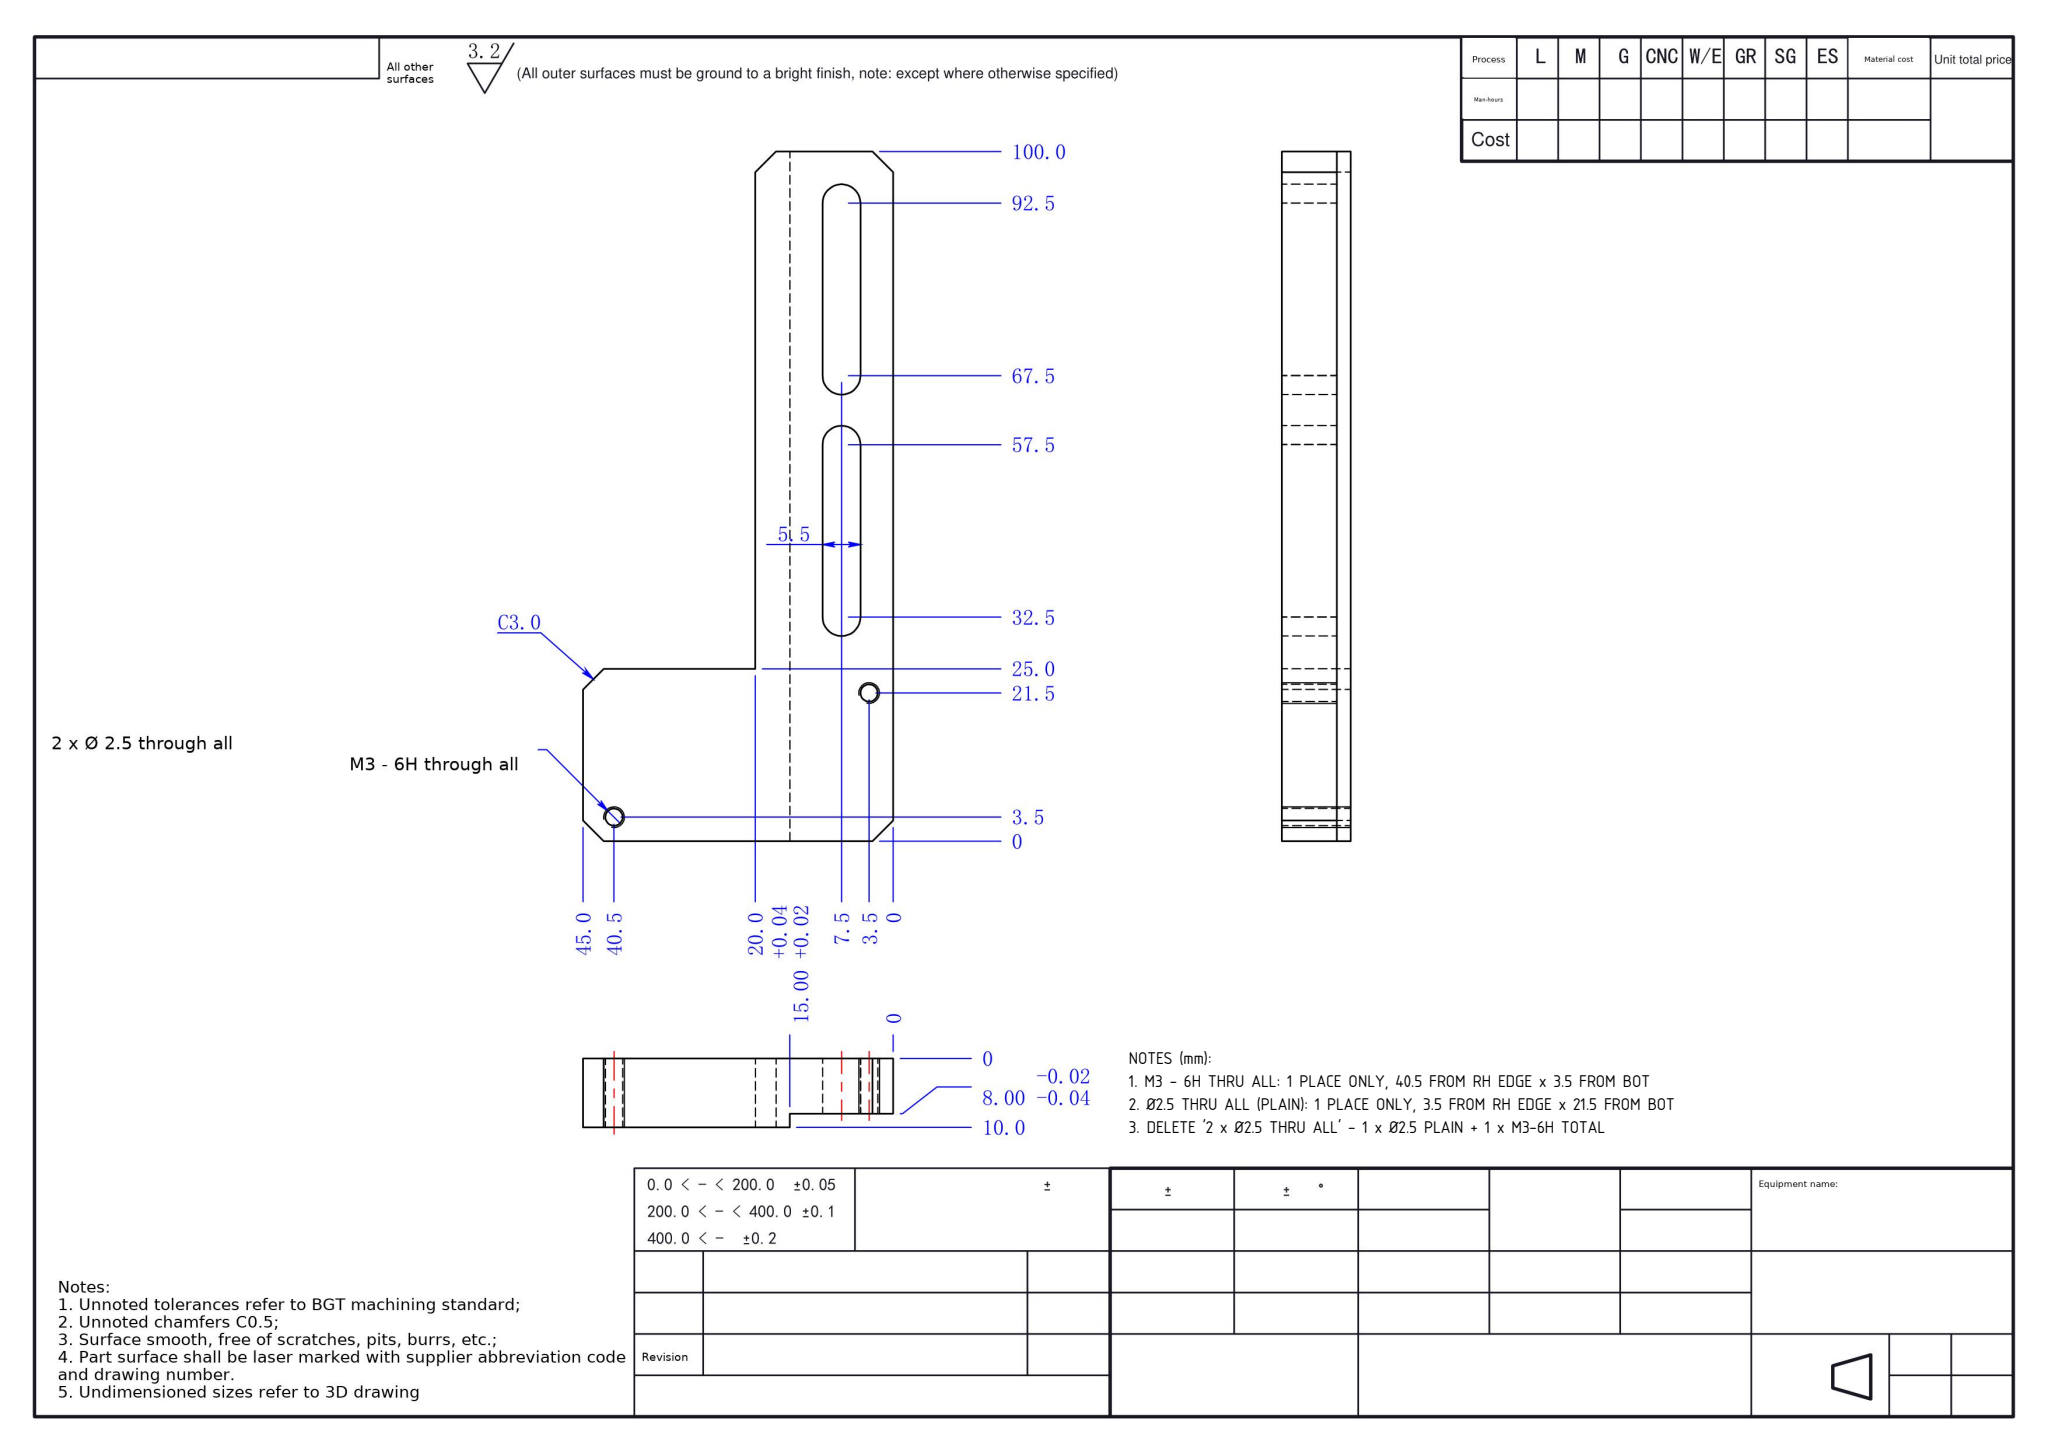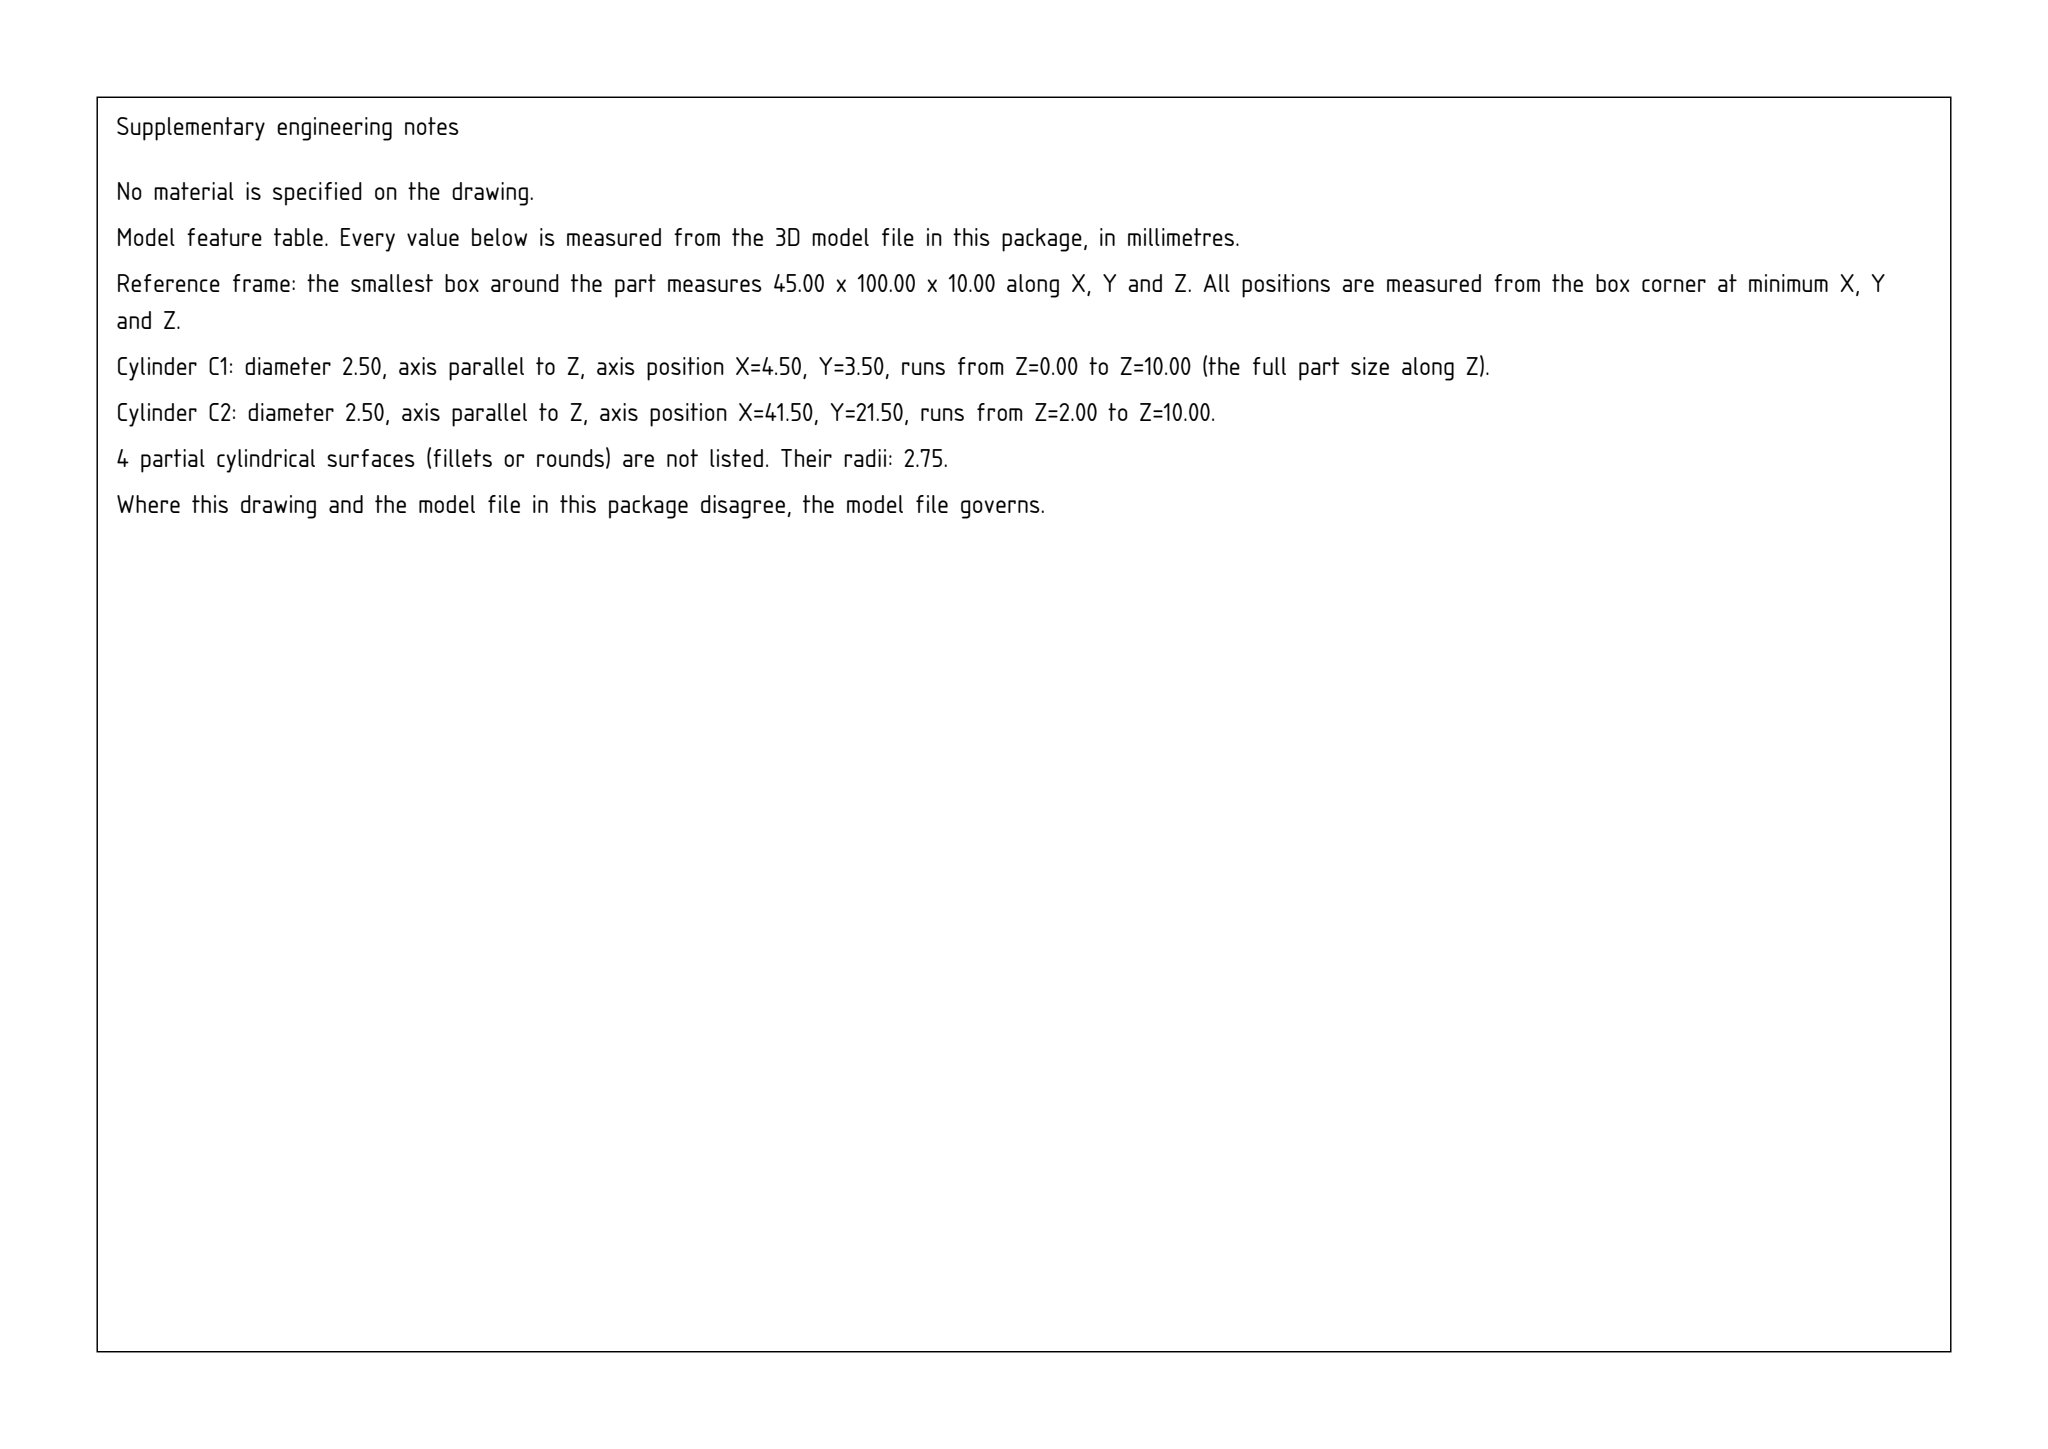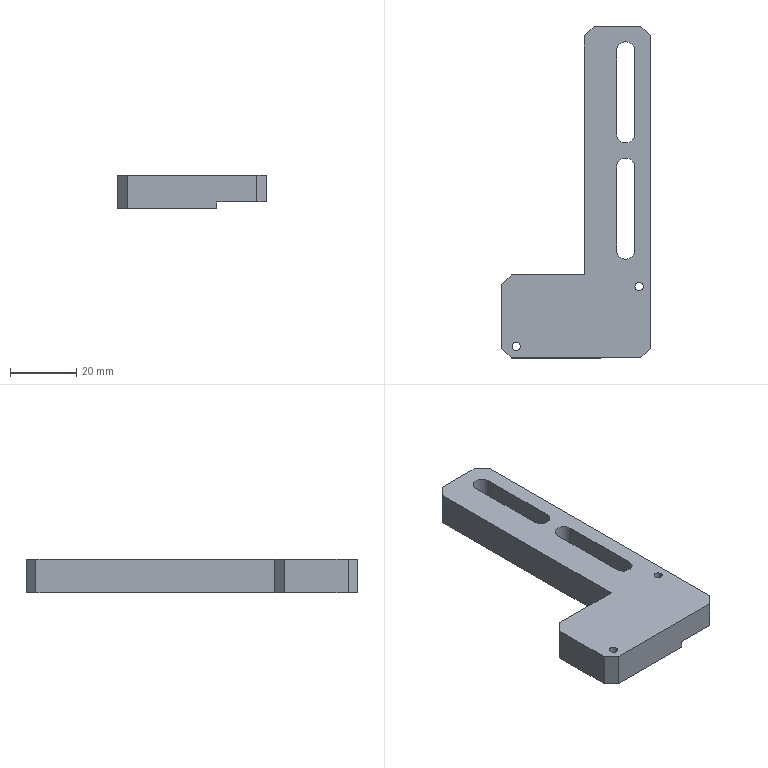Part | SolidWorks | mm | 1 solid | 27 faces | box 45 x 100 x 10 mm | volume 20375 mm3 | plane 19 | cylinder 8 | commonest cylinder face diameters 2.5 x4 5.5 x4
Drawing notes:
M3 - 6H THRU ALL: 1 PLACE ONLY, 40.5 FROM RH EDGE x 3.5 FROM BOT | from the solid: Ø2.5 z-axis cyl at (x=4.5, y=3.5), length 10 = full 10 thk; = 45.0-40.5 from RH edge datum (x=0 at right), 3.5 above y=0 bottom edge
Ø2.5 THRU ALL (PLAIN): 1 PLACE ONLY, 3.5 FROM RH EDGE x 21.5 FROM BOT | from the solid: Ø2.5 z-axis cyl at (x=41.5, y=21.5), length 8 = thk of 8.00 step region (z 2.0-10.0); = 45.0-41.5 from RH edge, 21.5 above bottom edge; only two Ø2.5 holes exist in model
DELETE '2 x Ø2.5 THRU ALL' - 1 x Ø2.5 PLAIN + 1 x M3-6H TOTAL | from the solid: Model contains exactly two Ø2.5 z-axis holes: (4.5,3.5) L10 and (41.5,21.5) L8
build123d program:
from build123d import *

# Parameters (mm, degrees)
SKETCH1_W           = 45
SKETCH1_H           = 100
BOSS_EXTRUDE1_DEPTH = 10
SKETCH2_W           = 25
SKETCH2_H           = 75
CUT_EXTRUDE1_DEPTH  = 111.114
SKETCH3_W           = 15
SKETCH3_H           = 100
CUT_EXTRUDE2_DEPTH  = 2
CHAMFER1_SIZE       = 3
CUT_EXTRUDE3_DEPTH  = 111.114
M3_TAPPED_HOLE1_D   = 2.5


with BuildPart() as part:
    # Sketch1 → Boss-Extrude1 (new body)
    with BuildSketch(Plane.XY):
        with Locations((22.5, 50)):
            Rectangle(SKETCH1_W, SKETCH1_H)
    extrude(amount=BOSS_EXTRUDE1_DEPTH)

    # Sketch2 → Cut-Extrude1 (cut, through all)
    with BuildSketch(Plane.XY.offset(10)):
        with Locations((12.5, 62.5)):
            Rectangle(SKETCH2_W, SKETCH2_H)
    extrude(amount=-CUT_EXTRUDE1_DEPTH, mode=Mode.SUBTRACT)

    # Sketch3 → Cut-Extrude2 (cut)
    with BuildSketch(Plane(origin=(0, 0, 0), x_dir=(-1, 0, 0), z_dir=(0, 0, -1))):
        with Locations((-37.5, 50)):
            Rectangle(SKETCH3_W, SKETCH3_H)
    extrude(amount=-CUT_EXTRUDE2_DEPTH, mode=Mode.SUBTRACT)

    # Chamfer1
    chamfer1_edges = [part.edges().sort_by_distance(p)[0] for p in [
        (0, 25, 5),
        (25, 100, 5),
        (45, 100, 6),
        (45, 0, 6),
        (0, 0, 5),
    ]]
    chamfer(chamfer1_edges, length=CHAMFER1_SIZE)

    # Sketch4 → Cut-Extrude3 (cut, through all)
    with BuildSketch(Plane.XY.offset(10)):
        with BuildLine():
            Line((40.25, 92.5), (40.25, 67.5))
            ThreePointArc((40.25, 67.5), (37.5, 64.75), (34.75, 67.5))
            Line((34.75, 67.5), (34.75, 92.5))
            ThreePointArc((34.75, 92.5), (37.5, 95.25), (40.25, 92.5))
        make_face()
        with BuildLine():
            Line((40.25, 57.5), (40.25, 32.5))
            ThreePointArc((40.25, 32.5), (37.5, 29.75), (34.75, 32.5))
            Line((34.75, 32.5), (34.75, 57.5))
            ThreePointArc((34.75, 57.5), (37.5, 60.25), (40.25, 57.5))
        make_face()
    extrude(amount=-CUT_EXTRUDE3_DEPTH, mode=Mode.SUBTRACT)

    # M3 Tapped Hole1 (through all)
    with Locations(Plane.XY.offset(10)):
        with Locations((4.5, 3.5), (41.5, 21.5)):
            Hole(M3_TAPPED_HOLE1_D / 2)


solid = part.part
STEP:
#1=CARTESIAN_POINT('',(3.25,3.5,0.));
#2=VERTEX_POINT('',#1);
#3=CARTESIAN_POINT('',(5.75,3.5,0.));
#4=VERTEX_POINT('',#3);
#5=CARTESIAN_POINT('',(4.5,3.5,0.));
#6=DIRECTION('',(0.,0.,1.));
#7=DIRECTION('',(1.,0.,0.));
#8=AXIS2_PLACEMENT_3D('',#5,#6,#7);
#9=CIRCLE('',#8,1.25);
#10=EDGE_CURVE('',#2,#4,#9,.T.);
#11=ORIENTED_EDGE('',*,*,#10,.F.);
#12=CARTESIAN_POINT('',(3.25,3.5,10.));
#13=VERTEX_POINT('',#12);
#14=CARTESIAN_POINT('',(3.25,3.5,10.));
#15=DIRECTION('',(0.,0.,1.));
#16=VECTOR('',#15,1000.);
#17=LINE('',#14,#16);
#18=EDGE_CURVE('',#2,#13,#17,.T.);
#19=ORIENTED_EDGE('',*,*,#18,.T.);
#20=CARTESIAN_POINT('',(5.75,3.5,10.));
#21=VERTEX_POINT('',#20);
#22=CARTESIAN_POINT('',(4.5,3.5,10.));
#23=DIRECTION('',(0.,0.,1.));
#24=DIRECTION('',(1.,0.,0.));
#25=AXIS2_PLACEMENT_3D('',#22,#23,#24);
#26=CIRCLE('',#25,1.25);
#27=EDGE_CURVE('',#13,#21,#26,.T.);
#28=ORIENTED_EDGE('',*,*,#27,.T.);
#29=CARTESIAN_POINT('',(5.75,3.5,10.));
#30=DIRECTION('',(0.,0.,1.));
#31=VECTOR('',#30,1000.);
#32=LINE('',#29,#31);
#33=EDGE_CURVE('',#4,#21,#32,.T.);
#34=ORIENTED_EDGE('',*,*,#33,.F.);
#35=EDGE_LOOP('',(#11,#19,#28,#34));
#36=FACE_OUTER_BOUND('',#35,.T.);
#37=CARTESIAN_POINT('',(4.5,3.5,10.));
#38=DIRECTION('',(0.,0.,1.));
#39=DIRECTION('',(1.,0.,0.));
#40=AXIS2_PLACEMENT_3D('',#37,#38,#39);
#41=CYLINDRICAL_SURFACE('',#40,1.25);
#42=ADVANCED_FACE('',(#36),#41,.F.);
#43=CARTESIAN_POINT('',(42.75,21.5,2.));
#44=VERTEX_POINT('',#43);
#45=CARTESIAN_POINT('',(40.25,21.5,2.));
#46=VERTEX_POINT('',#45);
#47=CARTESIAN_POINT('',(41.5,21.5,2.));
#48=DIRECTION('',(0.,0.,-1.));
#49=DIRECTION('',(-1.,0.,0.));
#50=AXIS2_PLACEMENT_3D('',#47,#48,#49);
#51=CIRCLE('',#50,1.25);
#52=EDGE_CURVE('',#44,#46,#51,.T.);
#53=ORIENTED_EDGE('',*,*,#52,.T.);
#54=CARTESIAN_POINT('',(40.25,21.5,10.));
#55=VERTEX_POINT('',#54);
#56=CARTESIAN_POINT('',(40.25,21.5,10.));
#57=DIRECTION('',(0.,0.,1.));
#58=VECTOR('',#57,1000.);
#59=LINE('',#56,#58);
#60=EDGE_CURVE('',#46,#55,#59,.T.);
#61=ORIENTED_EDGE('',*,*,#60,.T.);
#62=CARTESIAN_POINT('',(42.75,21.5,10.));
#63=VERTEX_POINT('',#62);
#64=CARTESIAN_POINT('',(41.5,21.5,10.));
#65=DIRECTION('',(0.,0.,1.));
#66=DIRECTION('',(1.,0.,0.));
#67=AXIS2_PLACEMENT_3D('',#64,#65,#66);
#68=CIRCLE('',#67,1.25);
#69=EDGE_CURVE('',#55,#63,#68,.T.);
#70=ORIENTED_EDGE('',*,*,#69,.T.);
#71=CARTESIAN_POINT('',(42.75,21.5,10.));
#72=DIRECTION('',(0.,0.,1.));
#73=VECTOR('',#72,1000.);
#74=LINE('',#71,#73);
#75=EDGE_CURVE('',#44,#63,#74,.T.);
#76=ORIENTED_EDGE('',*,*,#75,.F.);
#77=EDGE_LOOP('',(#53,#61,#70,#76));
#78=FACE_OUTER_BOUND('',#77,.T.);
#79=CARTESIAN_POINT('',(41.5,21.5,10.));
#80=DIRECTION('',(0.,0.,1.));
#81=DIRECTION('',(1.,0.,0.));
#82=AXIS2_PLACEMENT_3D('',#79,#80,#81);
#83=CYLINDRICAL_SURFACE('',#82,1.25);
#84=ADVANCED_FACE('',(#78),#83,.F.);
#85=CARTESIAN_POINT('',(41.5,21.5,10.));
#86=DIRECTION('',(0.,0.,1.));
#87=DIRECTION('',(1.,0.,0.));
#88=AXIS2_PLACEMENT_3D('',#85,#86,#87);
#89=CIRCLE('',#88,1.25);
#90=EDGE_CURVE('',#63,#55,#89,.T.);
#91=ORIENTED_EDGE('',*,*,#90,.F.);
#92=ORIENTED_EDGE('',*,*,#69,.F.);
#93=EDGE_LOOP('',(#91,#92));
#94=FACE_BOUND('',#93,.T.);
#95=CARTESIAN_POINT('',(34.75,57.5,10.));
#96=VERTEX_POINT('',#95);
#97=CARTESIAN_POINT('',(34.75,32.5,10.));
#98=VERTEX_POINT('',#97);
#99=CARTESIAN_POINT('',(34.75,57.5,10.));
#100=DIRECTION('',(0.,-1.,0.));
#101=VECTOR('',#100,1000.);
#102=LINE('',#99,#101);
#103=EDGE_CURVE('',#96,#98,#102,.T.);
#104=ORIENTED_EDGE('',*,*,#103,.F.);
#105=CARTESIAN_POINT('',(40.25,57.5,10.));
#106=VERTEX_POINT('',#105);
#107=CARTESIAN_POINT('',(37.5,57.5,10.));
#108=DIRECTION('',(0.,0.,1.));
#109=DIRECTION('',(1.,0.,0.));
#110=AXIS2_PLACEMENT_3D('',#107,#108,#109);
#111=CIRCLE('',#110,2.75);
#112=EDGE_CURVE('',#106,#96,#111,.T.);
#113=ORIENTED_EDGE('',*,*,#112,.F.);
#114=CARTESIAN_POINT('',(40.25,32.5,10.));
#115=VERTEX_POINT('',#114);
#116=CARTESIAN_POINT('',(40.25,57.5,10.));
#117=DIRECTION('',(-0.,1.,0.));
#118=VECTOR('',#117,1000.);
#119=LINE('',#116,#118);
#120=EDGE_CURVE('',#115,#106,#119,.T.);
#121=ORIENTED_EDGE('',*,*,#120,.F.);
#122=CARTESIAN_POINT('',(37.5,32.5,10.));
#123=DIRECTION('',(0.,0.,1.));
#124=DIRECTION('',(1.,0.,0.));
#125=AXIS2_PLACEMENT_3D('',#122,#123,#124);
#126=CIRCLE('',#125,2.75);
#127=EDGE_CURVE('',#98,#115,#126,.T.);
#128=ORIENTED_EDGE('',*,*,#127,.F.);
#129=EDGE_LOOP('',(#104,#113,#121,#128));
#130=FACE_BOUND('',#129,.T.);
#131=CARTESIAN_POINT('',(34.75,92.5,10.));
#132=VERTEX_POINT('',#131);
#133=CARTESIAN_POINT('',(34.75,67.5,10.));
#134=VERTEX_POINT('',#133);
#135=CARTESIAN_POINT('',(34.75,92.5,10.));
#136=DIRECTION('',(0.,-1.,0.));
#137=VECTOR('',#136,1000.);
#138=LINE('',#135,#137);
#139=EDGE_CURVE('',#132,#134,#138,.T.);
#140=ORIENTED_EDGE('',*,*,#139,.F.);
#141=CARTESIAN_POINT('',(40.25,92.5,10.));
#142=VERTEX_POINT('',#141);
#143=CARTESIAN_POINT('',(37.5,92.5,10.));
#144=DIRECTION('',(0.,0.,1.));
#145=DIRECTION('',(1.,0.,0.));
#146=AXIS2_PLACEMENT_3D('',#143,#144,#145);
#147=CIRCLE('',#146,2.75);
#148=EDGE_CURVE('',#142,#132,#147,.T.);
#149=ORIENTED_EDGE('',*,*,#148,.F.);
#150=CARTESIAN_POINT('',(40.25,67.5,10.));
#151=VERTEX_POINT('',#150);
#152=CARTESIAN_POINT('',(40.25,92.5,10.));
#153=DIRECTION('',(0.,1.,0.));
#154=VECTOR('',#153,1000.);
#155=LINE('',#152,#154);
#156=EDGE_CURVE('',#151,#142,#155,.T.);
#157=ORIENTED_EDGE('',*,*,#156,.F.);
#158=CARTESIAN_POINT('',(37.5,67.5,10.));
#159=DIRECTION('',(0.,0.,1.));
#160=DIRECTION('',(1.,0.,0.));
#161=AXIS2_PLACEMENT_3D('',#158,#159,#160);
#162=CIRCLE('',#161,2.75);
#163=EDGE_CURVE('',#134,#151,#162,.T.);
#164=ORIENTED_EDGE('',*,*,#163,.F.);
#165=EDGE_LOOP('',(#140,#149,#157,#164));
#166=FACE_BOUND('',#165,.T.);
#167=CARTESIAN_POINT('',(3.,0.,10.));
#168=VERTEX_POINT('',#167);
#169=CARTESIAN_POINT('',(42.,0.,10.));
#170=VERTEX_POINT('',#169);
#171=CARTESIAN_POINT('',(0.,0.,10.));
#172=DIRECTION('',(1.,0.,0.));
#173=VECTOR('',#172,1000.);
#174=LINE('',#171,#173);
#175=EDGE_CURVE('',#168,#170,#174,.T.);
#176=ORIENTED_EDGE('',*,*,#175,.T.);
#177=CARTESIAN_POINT('',(45.,3.,10.));
#178=VERTEX_POINT('',#177);
#179=CARTESIAN_POINT('',(45.,3.,10.));
#180=DIRECTION('',(0.7071,0.7071,0.));
#181=VECTOR('',#180,1000.);
#182=LINE('',#179,#181);
#183=EDGE_CURVE('',#170,#178,#182,.T.);
#184=ORIENTED_EDGE('',*,*,#183,.T.);
#185=CARTESIAN_POINT('',(45.,97.,10.));
#186=VERTEX_POINT('',#185);
#187=CARTESIAN_POINT('',(45.,0.,10.));
#188=DIRECTION('',(0.,1.,0.));
#189=VECTOR('',#188,1000.);
#190=LINE('',#187,#189);
#191=EDGE_CURVE('',#178,#186,#190,.T.);
#192=ORIENTED_EDGE('',*,*,#191,.T.);
#193=CARTESIAN_POINT('',(42.,100.,10.));
#194=VERTEX_POINT('',#193);
#195=CARTESIAN_POINT('',(42.,100.,10.));
#196=DIRECTION('',(-0.7071,0.7071,0.));
#197=VECTOR('',#196,1000.);
#198=LINE('',#195,#197);
#199=EDGE_CURVE('',#186,#194,#198,.T.);
#200=ORIENTED_EDGE('',*,*,#199,.T.);
#201=CARTESIAN_POINT('',(28.,100.,10.));
#202=VERTEX_POINT('',#201);
#203=CARTESIAN_POINT('',(0.,100.,10.));
#204=DIRECTION('',(-1.,0.,0.));
#205=VECTOR('',#204,1000.);
#206=LINE('',#203,#205);
#207=EDGE_CURVE('',#194,#202,#206,.T.);
#208=ORIENTED_EDGE('',*,*,#207,.T.);
#209=CARTESIAN_POINT('',(25.,97.,10.));
#210=VERTEX_POINT('',#209);
#211=CARTESIAN_POINT('',(28.,100.,10.));
#212=DIRECTION('',(-0.7071,-0.7071,0.));
#213=VECTOR('',#212,1000.);
#214=LINE('',#211,#213);
#215=EDGE_CURVE('',#202,#210,#214,.T.);
#216=ORIENTED_EDGE('',*,*,#215,.T.);
#217=CARTESIAN_POINT('',(25.,25.,10.));
#218=VERTEX_POINT('',#217);
#219=CARTESIAN_POINT('',(25.,100.,10.));
#220=DIRECTION('',(-0.,1.,0.));
#221=VECTOR('',#220,1000.);
#222=LINE('',#219,#221);
#223=EDGE_CURVE('',#218,#210,#222,.T.);
#224=ORIENTED_EDGE('',*,*,#223,.F.);
#225=CARTESIAN_POINT('',(3.,25.,10.));
#226=VERTEX_POINT('',#225);
#227=CARTESIAN_POINT('',(0.,25.,10.));
#228=DIRECTION('',(1.,0.,0.));
#229=VECTOR('',#228,1000.);
#230=LINE('',#227,#229);
#231=EDGE_CURVE('',#226,#218,#230,.T.);
#232=ORIENTED_EDGE('',*,*,#231,.F.);
#233=CARTESIAN_POINT('',(0.,22.,10.));
#234=VERTEX_POINT('',#233);
#235=CARTESIAN_POINT('',(3.,25.,10.));
#236=DIRECTION('',(-0.7071,-0.7071,0.));
#237=VECTOR('',#236,1000.);
#238=LINE('',#235,#237);
#239=EDGE_CURVE('',#226,#234,#238,.T.);
#240=ORIENTED_EDGE('',*,*,#239,.T.);
#241=CARTESIAN_POINT('',(0.,3.,10.));
#242=VERTEX_POINT('',#241);
#243=CARTESIAN_POINT('',(0.,0.,10.));
#244=DIRECTION('',(0.,-1.,0.));
#245=VECTOR('',#244,1000.);
#246=LINE('',#243,#245);
#247=EDGE_CURVE('',#234,#242,#246,.T.);
#248=ORIENTED_EDGE('',*,*,#247,.T.);
#249=CARTESIAN_POINT('',(3.,0.,10.));
#250=DIRECTION('',(0.7071,-0.7071,0.));
#251=VECTOR('',#250,1000.);
#252=LINE('',#249,#251);
#253=EDGE_CURVE('',#242,#168,#252,.T.);
#254=ORIENTED_EDGE('',*,*,#253,.T.);
#255=EDGE_LOOP('',(#176,#184,#192,#200,#208,#216,#224,#232,#240,#248,#254));
#256=FACE_OUTER_BOUND('',#255,.T.);
#257=CARTESIAN_POINT('',(4.5,3.5,10.));
#258=DIRECTION('',(0.,0.,1.));
#259=DIRECTION('',(1.,0.,0.));
#260=AXIS2_PLACEMENT_3D('',#257,#258,#259);
#261=CIRCLE('',#260,1.25);
#262=EDGE_CURVE('',#21,#13,#261,.T.);
#263=ORIENTED_EDGE('',*,*,#262,.F.);
#264=ORIENTED_EDGE('',*,*,#27,.F.);
#265=EDGE_LOOP('',(#263,#264));
#266=FACE_BOUND('',#265,.T.);
#267=CARTESIAN_POINT('',(0.,0.,10.));
#268=DIRECTION('',(0.,0.,-1.));
#269=DIRECTION('',(-1.,0.,0.));
#270=AXIS2_PLACEMENT_3D('',#267,#268,#269);
#271=PLANE('',#270);
#272=ADVANCED_FACE('',(#94,#130,#166,#256,#266),#271,.F.);
#273=ORIENTED_EDGE('',*,*,#191,.F.);
#274=CARTESIAN_POINT('',(45.,3.,2.));
#275=VERTEX_POINT('',#274);
#276=CARTESIAN_POINT('',(45.,3.,10.));
#277=DIRECTION('',(0.,0.,-1.));
#278=VECTOR('',#277,1000.);
#279=LINE('',#276,#278);
#280=EDGE_CURVE('',#178,#275,#279,.T.);
#281=ORIENTED_EDGE('',*,*,#280,.T.);
#282=CARTESIAN_POINT('',(45.,97.,2.));
#283=VERTEX_POINT('',#282);
#284=CARTESIAN_POINT('',(45.,100.,2.));
#285=DIRECTION('',(0.,-1.,0.));
#286=VECTOR('',#285,1000.);
#287=LINE('',#284,#286);
#288=EDGE_CURVE('',#283,#275,#287,.T.);
#289=ORIENTED_EDGE('',*,*,#288,.F.);
#290=CARTESIAN_POINT('',(45.,97.,10.));
#291=DIRECTION('',(0.,0.,1.));
#292=VECTOR('',#291,1000.);
#293=LINE('',#290,#292);
#294=EDGE_CURVE('',#283,#186,#293,.T.);
#295=ORIENTED_EDGE('',*,*,#294,.T.);
#296=EDGE_LOOP('',(#273,#281,#289,#295));
#297=FACE_OUTER_BOUND('',#296,.T.);
#298=CARTESIAN_POINT('',(45.,0.,10.));
#299=DIRECTION('',(-1.,0.,0.));
#300=DIRECTION('',(0.,0.,1.));
#301=AXIS2_PLACEMENT_3D('',#298,#299,#300);
#302=PLANE('',#301);
#303=ADVANCED_FACE('',(#297),#302,.F.);
#304=CARTESIAN_POINT('',(0.,22.,0.));
#305=VERTEX_POINT('',#304);
#306=CARTESIAN_POINT('',(0.,3.,0.));
#307=VERTEX_POINT('',#306);
#308=CARTESIAN_POINT('',(0.,0.,0.));
#309=DIRECTION('',(0.,-1.,0.));
#310=VECTOR('',#309,1000.);
#311=LINE('',#308,#310);
#312=EDGE_CURVE('',#305,#307,#311,.T.);
#313=ORIENTED_EDGE('',*,*,#312,.T.);
#314=CARTESIAN_POINT('',(0.,3.,10.));
#315=DIRECTION('',(0.,0.,1.));
#316=VECTOR('',#315,1000.);
#317=LINE('',#314,#316);
#318=EDGE_CURVE('',#307,#242,#317,.T.);
#319=ORIENTED_EDGE('',*,*,#318,.T.);
#320=ORIENTED_EDGE('',*,*,#247,.F.);
#321=CARTESIAN_POINT('',(0.,22.,10.));
#322=DIRECTION('',(0.,0.,-1.));
#323=VECTOR('',#322,1000.);
#324=LINE('',#321,#323);
#325=EDGE_CURVE('',#234,#305,#324,.T.);
#326=ORIENTED_EDGE('',*,*,#325,.T.);
#327=EDGE_LOOP('',(#313,#319,#320,#326));
#328=FACE_OUTER_BOUND('',#327,.T.);
#329=CARTESIAN_POINT('',(0.,0.,10.));
#330=DIRECTION('',(1.,0.,0.));
#331=DIRECTION('',(0.,0.,-1.));
#332=AXIS2_PLACEMENT_3D('',#329,#330,#331);
#333=PLANE('',#332);
#334=ADVANCED_FACE('',(#328),#333,.F.);
#335=CARTESIAN_POINT('',(42.,0.,2.));
#336=VERTEX_POINT('',#335);
#337=CARTESIAN_POINT('',(30.,0.,2.));
#338=VERTEX_POINT('',#337);
#339=CARTESIAN_POINT('',(45.,0.,2.));
#340=DIRECTION('',(-1.,0.,0.));
#341=VECTOR('',#340,1000.);
#342=LINE('',#339,#341);
#343=EDGE_CURVE('',#336,#338,#342,.T.);
#344=ORIENTED_EDGE('',*,*,#343,.F.);
#345=CARTESIAN_POINT('',(42.,0.,10.));
#346=DIRECTION('',(0.,0.,1.));
#347=VECTOR('',#346,1000.);
#348=LINE('',#345,#347);
#349=EDGE_CURVE('',#336,#170,#348,.T.);
#350=ORIENTED_EDGE('',*,*,#349,.T.);
#351=ORIENTED_EDGE('',*,*,#175,.F.);
#352=CARTESIAN_POINT('',(3.,0.,0.));
#353=VERTEX_POINT('',#352);
#354=CARTESIAN_POINT('',(3.,0.,10.));
#355=DIRECTION('',(0.,0.,-1.));
#356=VECTOR('',#355,1000.);
#357=LINE('',#354,#356);
#358=EDGE_CURVE('',#168,#353,#357,.T.);
#359=ORIENTED_EDGE('',*,*,#358,.T.);
#360=CARTESIAN_POINT('',(30.,0.,0.));
#361=VERTEX_POINT('',#360);
#362=CARTESIAN_POINT('',(0.,0.,0.));
#363=DIRECTION('',(1.,0.,0.));
#364=VECTOR('',#363,1000.);
#365=LINE('',#362,#364);
#366=EDGE_CURVE('',#353,#361,#365,.T.);
#367=ORIENTED_EDGE('',*,*,#366,.T.);
#368=CARTESIAN_POINT('',(30.,0.,2.));
#369=DIRECTION('',(0.,0.,-1.));
#370=VECTOR('',#369,1000.);
#371=LINE('',#368,#370);
#372=EDGE_CURVE('',#338,#361,#371,.T.);
#373=ORIENTED_EDGE('',*,*,#372,.F.);
#374=EDGE_LOOP('',(#344,#350,#351,#359,#367,#373));
#375=FACE_OUTER_BOUND('',#374,.T.);
#376=CARTESIAN_POINT('',(0.,0.,10.));
#377=DIRECTION('',(0.,1.,0.));
#378=DIRECTION('',(0.,0.,1.));
#379=AXIS2_PLACEMENT_3D('',#376,#377,#378);
#380=PLANE('',#379);
#381=ADVANCED_FACE('',(#375),#380,.F.);
#382=CARTESIAN_POINT('',(30.,100.,0.));
#383=VERTEX_POINT('',#382);
#384=CARTESIAN_POINT('',(28.,100.,0.));
#385=VERTEX_POINT('',#384);
#386=CARTESIAN_POINT('',(0.,100.,0.));
#387=DIRECTION('',(-1.,0.,0.));
#388=VECTOR('',#387,1000.);
#389=LINE('',#386,#388);
#390=EDGE_CURVE('',#383,#385,#389,.T.);
#391=ORIENTED_EDGE('',*,*,#390,.T.);
#392=CARTESIAN_POINT('',(28.,100.,10.));
#393=DIRECTION('',(0.,0.,1.));
#394=VECTOR('',#393,1000.);
#395=LINE('',#392,#394);
#396=EDGE_CURVE('',#385,#202,#395,.T.);
#397=ORIENTED_EDGE('',*,*,#396,.T.);
#398=ORIENTED_EDGE('',*,*,#207,.F.);
#399=CARTESIAN_POINT('',(42.,100.,2.));
#400=VERTEX_POINT('',#399);
#401=CARTESIAN_POINT('',(42.,100.,10.));
#402=DIRECTION('',(0.,0.,-1.));
#403=VECTOR('',#402,1000.);
#404=LINE('',#401,#403);
#405=EDGE_CURVE('',#194,#400,#404,.T.);
#406=ORIENTED_EDGE('',*,*,#405,.T.);
#407=CARTESIAN_POINT('',(30.,100.,2.));
#408=VERTEX_POINT('',#407);
#409=CARTESIAN_POINT('',(45.,100.,2.));
#410=DIRECTION('',(1.,0.,0.));
#411=VECTOR('',#410,1000.);
#412=LINE('',#409,#411);
#413=EDGE_CURVE('',#408,#400,#412,.T.);
#414=ORIENTED_EDGE('',*,*,#413,.F.);
#415=CARTESIAN_POINT('',(30.,100.,2.));
#416=DIRECTION('',(0.,0.,-1.));
#417=VECTOR('',#416,1000.);
#418=LINE('',#415,#417);
#419=EDGE_CURVE('',#408,#383,#418,.T.);
#420=ORIENTED_EDGE('',*,*,#419,.T.);
#421=EDGE_LOOP('',(#391,#397,#398,#406,#414,#420));
#422=FACE_OUTER_BOUND('',#421,.T.);
#423=CARTESIAN_POINT('',(0.,100.,10.));
#424=DIRECTION('',(0.,-1.,0.));
#425=DIRECTION('',(0.,0.,-1.));
#426=AXIS2_PLACEMENT_3D('',#423,#424,#425);
#427=PLANE('',#426);
#428=ADVANCED_FACE('',(#422),#427,.F.);
#429=CARTESIAN_POINT('',(4.5,3.5,0.));
#430=DIRECTION('',(0.,0.,1.));
#431=DIRECTION('',(1.,0.,0.));
#432=AXIS2_PLACEMENT_3D('',#429,#430,#431);
#433=CIRCLE('',#432,1.25);
#434=EDGE_CURVE('',#4,#2,#433,.T.);
#435=ORIENTED_EDGE('',*,*,#434,.T.);
#436=ORIENTED_EDGE('',*,*,#10,.T.);
#437=EDGE_LOOP('',(#435,#436));
#438=FACE_BOUND('',#437,.T.);
#439=ORIENTED_EDGE('',*,*,#366,.F.);
#440=CARTESIAN_POINT('',(1.5,1.5,0.));
#441=DIRECTION('',(-0.7071,0.7071,0.));
#442=VECTOR('',#441,1000.);
#443=LINE('',#440,#442);
#444=EDGE_CURVE('',#353,#307,#443,.T.);
#445=ORIENTED_EDGE('',*,*,#444,.T.);
#446=ORIENTED_EDGE('',*,*,#312,.F.);
#447=CARTESIAN_POINT('',(3.,25.,0.));
#448=VERTEX_POINT('',#447);
#449=CARTESIAN_POINT('',(-11.,11.,0.));
#450=DIRECTION('',(0.7071,0.7071,0.));
#451=VECTOR('',#450,1000.);
#452=LINE('',#449,#451);
#453=EDGE_CURVE('',#305,#448,#452,.T.);
#454=ORIENTED_EDGE('',*,*,#453,.T.);
#455=CARTESIAN_POINT('',(25.,25.,0.));
#456=VERTEX_POINT('',#455);
#457=CARTESIAN_POINT('',(0.,25.,0.));
#458=DIRECTION('',(1.,0.,0.));
#459=VECTOR('',#458,1000.);
#460=LINE('',#457,#459);
#461=EDGE_CURVE('',#448,#456,#460,.T.);
#462=ORIENTED_EDGE('',*,*,#461,.T.);
#463=CARTESIAN_POINT('',(25.,97.,0.));
#464=VERTEX_POINT('',#463);
#465=CARTESIAN_POINT('',(25.,100.,0.));
#466=DIRECTION('',(-0.,1.,0.));
#467=VECTOR('',#466,1000.);
#468=LINE('',#465,#467);
#469=EDGE_CURVE('',#456,#464,#468,.T.);
#470=ORIENTED_EDGE('',*,*,#469,.T.);
#471=CARTESIAN_POINT('',(-36.,36.,0.));
#472=DIRECTION('',(0.7071,0.7071,0.));
#473=VECTOR('',#472,1000.);
#474=LINE('',#471,#473);
#475=EDGE_CURVE('',#464,#385,#474,.T.);
#476=ORIENTED_EDGE('',*,*,#475,.T.);
#477=ORIENTED_EDGE('',*,*,#390,.F.);
#478=CARTESIAN_POINT('',(30.,100.,0.));
#479=DIRECTION('',(0.,1.,0.));
#480=VECTOR('',#479,1000.);
#481=LINE('',#478,#480);
#482=EDGE_CURVE('',#361,#383,#481,.T.);
#483=ORIENTED_EDGE('',*,*,#482,.F.);
#484=EDGE_LOOP('',(#439,#445,#446,#454,#462,#470,#476,#477,#483));
#485=FACE_OUTER_BOUND('',#484,.T.);
#486=CARTESIAN_POINT('',(0.,0.,0.));
#487=DIRECTION('',(0.,0.,-1.));
#488=DIRECTION('',(-1.,0.,0.));
#489=AXIS2_PLACEMENT_3D('',#486,#487,#488);
#490=PLANE('',#489);
#491=ADVANCED_FACE('',(#438,#485),#490,.T.);
#492=ORIENTED_EDGE('',*,*,#223,.T.);
#493=CARTESIAN_POINT('',(25.,97.,0.));
#494=DIRECTION('',(0.,0.,-1.));
#495=VECTOR('',#494,1000.);
#496=LINE('',#493,#495);
#497=EDGE_CURVE('',#210,#464,#496,.T.);
#498=ORIENTED_EDGE('',*,*,#497,.T.);
#499=ORIENTED_EDGE('',*,*,#469,.F.);
#500=CARTESIAN_POINT('',(25.,25.,0.));
#501=DIRECTION('',(0.,0.,1.));
#502=VECTOR('',#501,1000.);
#503=LINE('',#500,#502);
#504=EDGE_CURVE('',#456,#218,#503,.T.);
#505=ORIENTED_EDGE('',*,*,#504,.T.);
#506=EDGE_LOOP('',(#492,#498,#499,#505));
#507=FACE_OUTER_BOUND('',#506,.T.);
#508=CARTESIAN_POINT('',(25.,100.,0.));
#509=DIRECTION('',(1.,0.,0.));
#510=DIRECTION('',(-0.,1.,0.));
#511=AXIS2_PLACEMENT_3D('',#508,#509,#510);
#512=PLANE('',#511);
#513=ADVANCED_FACE('',(#507),#512,.F.);
#514=ORIENTED_EDGE('',*,*,#461,.F.);
#515=CARTESIAN_POINT('',(3.,25.,0.));
#516=DIRECTION('',(0.,0.,1.));
#517=VECTOR('',#516,1000.);
#518=LINE('',#515,#517);
#519=EDGE_CURVE('',#448,#226,#518,.T.);
#520=ORIENTED_EDGE('',*,*,#519,.T.);
#521=ORIENTED_EDGE('',*,*,#231,.T.);
#522=ORIENTED_EDGE('',*,*,#504,.F.);
#523=EDGE_LOOP('',(#514,#520,#521,#522));
#524=FACE_OUTER_BOUND('',#523,.T.);
#525=CARTESIAN_POINT('',(0.,25.,0.));
#526=DIRECTION('',(0.,-1.,0.));
#527=DIRECTION('',(0.,0.,-1.));
#528=AXIS2_PLACEMENT_3D('',#525,#526,#527);
#529=PLANE('',#528);
#530=ADVANCED_FACE('',(#524),#529,.F.);
#531=ORIENTED_EDGE('',*,*,#482,.T.);
#532=ORIENTED_EDGE('',*,*,#419,.F.);
#533=CARTESIAN_POINT('',(30.,100.,2.));
#534=DIRECTION('',(0.,1.,0.));
#535=VECTOR('',#534,1000.);
#536=LINE('',#533,#535);
#537=EDGE_CURVE('',#338,#408,#536,.T.);
#538=ORIENTED_EDGE('',*,*,#537,.F.);
#539=ORIENTED_EDGE('',*,*,#372,.T.);
#540=EDGE_LOOP('',(#531,#532,#538,#539));
#541=FACE_OUTER_BOUND('',#540,.T.);
#542=CARTESIAN_POINT('',(30.,100.,2.));
#543=DIRECTION('',(-1.,0.,0.));
#544=DIRECTION('',(-0.,-1.,0.));
#545=AXIS2_PLACEMENT_3D('',#542,#543,#544);
#546=PLANE('',#545);
#547=ADVANCED_FACE('',(#541),#546,.F.);
#548=ORIENTED_EDGE('',*,*,#52,.F.);
#549=CARTESIAN_POINT('',(41.5,21.5,2.));
#550=DIRECTION('',(0.,0.,-1.));
#551=DIRECTION('',(-1.,0.,0.));
#552=AXIS2_PLACEMENT_3D('',#549,#550,#551);
#553=CIRCLE('',#552,1.25);
#554=EDGE_CURVE('',#46,#44,#553,.T.);
#555=ORIENTED_EDGE('',*,*,#554,.F.);
#556=EDGE_LOOP('',(#548,#555));
#557=FACE_BOUND('',#556,.T.);
#558=CARTESIAN_POINT('',(34.75,57.5,2.));
#559=VERTEX_POINT('',#558);
#560=CARTESIAN_POINT('',(40.25,57.5,2.));
#561=VERTEX_POINT('',#560);
#562=CARTESIAN_POINT('',(37.5,57.5,2.));
#563=DIRECTION('',(0.,0.,-1.));
#564=DIRECTION('',(-1.,0.,0.));
#565=AXIS2_PLACEMENT_3D('',#562,#563,#564);
#566=CIRCLE('',#565,2.75);
#567=EDGE_CURVE('',#559,#561,#566,.T.);
#568=ORIENTED_EDGE('',*,*,#567,.F.);
#569=CARTESIAN_POINT('',(34.75,32.5,2.));
#570=VERTEX_POINT('',#569);
#571=CARTESIAN_POINT('',(34.75,0.,2.));
#572=DIRECTION('',(-0.,1.,0.));
#573=VECTOR('',#572,1000.);
#574=LINE('',#571,#573);
#575=EDGE_CURVE('',#570,#559,#574,.T.);
#576=ORIENTED_EDGE('',*,*,#575,.F.);
#577=CARTESIAN_POINT('',(40.25,32.5,2.));
#578=VERTEX_POINT('',#577);
#579=CARTESIAN_POINT('',(37.5,32.5,2.));
#580=DIRECTION('',(0.,0.,-1.));
#581=DIRECTION('',(-1.,0.,0.));
#582=AXIS2_PLACEMENT_3D('',#579,#580,#581);
#583=CIRCLE('',#582,2.75);
#584=EDGE_CURVE('',#578,#570,#583,.T.);
#585=ORIENTED_EDGE('',*,*,#584,.F.);
#586=CARTESIAN_POINT('',(40.25,0.,2.));
#587=DIRECTION('',(0.,-1.,0.));
#588=VECTOR('',#587,1000.);
#589=LINE('',#586,#588);
#590=EDGE_CURVE('',#561,#578,#589,.T.);
#591=ORIENTED_EDGE('',*,*,#590,.F.);
#592=EDGE_LOOP('',(#568,#576,#585,#591));
#593=FACE_BOUND('',#592,.T.);
#594=CARTESIAN_POINT('',(34.75,92.5,2.));
#595=VERTEX_POINT('',#594);
#596=CARTESIAN_POINT('',(40.25,92.5,2.));
#597=VERTEX_POINT('',#596);
#598=CARTESIAN_POINT('',(37.5,92.5,2.));
#599=DIRECTION('',(0.,0.,-1.));
#600=DIRECTION('',(-1.,0.,0.));
#601=AXIS2_PLACEMENT_3D('',#598,#599,#600);
#602=CIRCLE('',#601,2.75);
#603=EDGE_CURVE('',#595,#597,#602,.T.);
#604=ORIENTED_EDGE('',*,*,#603,.F.);
#605=CARTESIAN_POINT('',(34.75,67.5,2.));
#606=VERTEX_POINT('',#605);
#607=CARTESIAN_POINT('',(34.75,0.,2.));
#608=DIRECTION('',(0.,1.,0.));
#609=VECTOR('',#608,1000.);
#610=LINE('',#607,#609);
#611=EDGE_CURVE('',#606,#595,#610,.T.);
#612=ORIENTED_EDGE('',*,*,#611,.F.);
#613=CARTESIAN_POINT('',(40.25,67.5,2.));
#614=VERTEX_POINT('',#613);
#615=CARTESIAN_POINT('',(37.5,67.5,2.));
#616=DIRECTION('',(0.,0.,-1.));
#617=DIRECTION('',(-1.,0.,0.));
#618=AXIS2_PLACEMENT_3D('',#615,#616,#617);
#619=CIRCLE('',#618,2.75);
#620=EDGE_CURVE('',#614,#606,#619,.T.);
#621=ORIENTED_EDGE('',*,*,#620,.F.);
#622=CARTESIAN_POINT('',(40.25,0.,2.));
#623=DIRECTION('',(0.,-1.,0.));
#624=VECTOR('',#623,1000.);
#625=LINE('',#622,#624);
#626=EDGE_CURVE('',#597,#614,#625,.T.);
#627=ORIENTED_EDGE('',*,*,#626,.F.);
#628=EDGE_LOOP('',(#604,#612,#621,#627));
#629=FACE_BOUND('',#628,.T.);
#630=ORIENTED_EDGE('',*,*,#288,.T.);
#631=CARTESIAN_POINT('',(21.,-21.,2.));
#632=DIRECTION('',(-0.7071,-0.7071,0.));
#633=VECTOR('',#632,1000.);
#634=LINE('',#631,#633);
#635=EDGE_CURVE('',#275,#336,#634,.T.);
#636=ORIENTED_EDGE('',*,*,#635,.T.);
#637=ORIENTED_EDGE('',*,*,#343,.T.);
#638=ORIENTED_EDGE('',*,*,#537,.T.);
#639=ORIENTED_EDGE('',*,*,#413,.T.);
#640=CARTESIAN_POINT('',(71.,71.,2.));
#641=DIRECTION('',(0.7071,-0.7071,0.));
#642=VECTOR('',#641,1000.);
#643=LINE('',#640,#642);
#644=EDGE_CURVE('',#400,#283,#643,.T.);
#645=ORIENTED_EDGE('',*,*,#644,.T.);
#646=EDGE_LOOP('',(#630,#636,#637,#638,#639,#645));
#647=FACE_OUTER_BOUND('',#646,.T.);
#648=CARTESIAN_POINT('',(0.,0.,2.));
#649=DIRECTION('',(0.,0.,-1.));
#650=DIRECTION('',(-1.,0.,0.));
#651=AXIS2_PLACEMENT_3D('',#648,#649,#650);
#652=PLANE('',#651);
#653=ADVANCED_FACE('',(#557,#593,#629,#647),#652,.T.);
#654=ORIENTED_EDGE('',*,*,#183,.F.);
#655=ORIENTED_EDGE('',*,*,#349,.F.);
#656=ORIENTED_EDGE('',*,*,#635,.F.);
#657=ORIENTED_EDGE('',*,*,#280,.F.);
#658=EDGE_LOOP('',(#654,#655,#656,#657));
#659=FACE_OUTER_BOUND('',#658,.T.);
#660=CARTESIAN_POINT('',(45.,3.,10.));
#661=DIRECTION('',(-0.7071,0.7071,0.));
#662=DIRECTION('',(0.,0.,-1.));
#663=AXIS2_PLACEMENT_3D('',#660,#661,#662);
#664=PLANE('',#663);
#665=ADVANCED_FACE('',(#659),#664,.F.);
#666=ORIENTED_EDGE('',*,*,#253,.F.);
#667=ORIENTED_EDGE('',*,*,#318,.F.);
#668=ORIENTED_EDGE('',*,*,#444,.F.);
#669=ORIENTED_EDGE('',*,*,#358,.F.);
#670=EDGE_LOOP('',(#666,#667,#668,#669));
#671=FACE_OUTER_BOUND('',#670,.T.);
#672=CARTESIAN_POINT('',(3.,0.,10.));
#673=DIRECTION('',(0.7071,0.7071,0.));
#674=DIRECTION('',(0.,0.,-1.));
#675=AXIS2_PLACEMENT_3D('',#672,#673,#674);
#676=PLANE('',#675);
#677=ADVANCED_FACE('',(#671),#676,.F.);
#678=ORIENTED_EDGE('',*,*,#453,.F.);
#679=ORIENTED_EDGE('',*,*,#325,.F.);
#680=ORIENTED_EDGE('',*,*,#239,.F.);
#681=ORIENTED_EDGE('',*,*,#519,.F.);
#682=EDGE_LOOP('',(#678,#679,#680,#681));
#683=FACE_OUTER_BOUND('',#682,.T.);
#684=CARTESIAN_POINT('',(3.,25.,0.));
#685=DIRECTION('',(0.7071,-0.7071,0.));
#686=DIRECTION('',(0.,0.,1.));
#687=AXIS2_PLACEMENT_3D('',#684,#685,#686);
#688=PLANE('',#687);
#689=ADVANCED_FACE('',(#683),#688,.F.);
#690=ORIENTED_EDGE('',*,*,#475,.F.);
#691=ORIENTED_EDGE('',*,*,#497,.F.);
#692=ORIENTED_EDGE('',*,*,#215,.F.);
#693=ORIENTED_EDGE('',*,*,#396,.F.);
#694=EDGE_LOOP('',(#690,#691,#692,#693));
#695=FACE_OUTER_BOUND('',#694,.T.);
#696=CARTESIAN_POINT('',(28.,100.,10.));
#697=DIRECTION('',(0.7071,-0.7071,0.));
#698=DIRECTION('',(0.,0.,1.));
#699=AXIS2_PLACEMENT_3D('',#696,#697,#698);
#700=PLANE('',#699);
#701=ADVANCED_FACE('',(#695),#700,.F.);
#702=ORIENTED_EDGE('',*,*,#199,.F.);
#703=ORIENTED_EDGE('',*,*,#294,.F.);
#704=ORIENTED_EDGE('',*,*,#644,.F.);
#705=ORIENTED_EDGE('',*,*,#405,.F.);
#706=EDGE_LOOP('',(#702,#703,#704,#705));
#707=FACE_OUTER_BOUND('',#706,.T.);
#708=CARTESIAN_POINT('',(42.,100.,10.));
#709=DIRECTION('',(-0.7071,-0.7071,0.));
#710=DIRECTION('',(0.,0.,-1.));
#711=AXIS2_PLACEMENT_3D('',#708,#709,#710);
#712=PLANE('',#711);
#713=ADVANCED_FACE('',(#707),#712,.F.);
#714=ORIENTED_EDGE('',*,*,#603,.T.);
#715=CARTESIAN_POINT('',(40.25,92.5,0.));
#716=DIRECTION('',(0.,0.,1.));
#717=VECTOR('',#716,1000.);
#718=LINE('',#715,#717);
#719=EDGE_CURVE('',#597,#142,#718,.T.);
#720=ORIENTED_EDGE('',*,*,#719,.T.);
#721=ORIENTED_EDGE('',*,*,#148,.T.);
#722=CARTESIAN_POINT('',(34.75,92.5,0.));
#723=DIRECTION('',(0.,0.,1.));
#724=VECTOR('',#723,1000.);
#725=LINE('',#722,#724);
#726=EDGE_CURVE('',#595,#132,#725,.T.);
#727=ORIENTED_EDGE('',*,*,#726,.F.);
#728=EDGE_LOOP('',(#714,#720,#721,#727));
#729=FACE_OUTER_BOUND('',#728,.T.);
#730=CARTESIAN_POINT('',(37.5,92.5,0.));
#731=DIRECTION('',(0.,0.,1.));
#732=DIRECTION('',(1.,0.,0.));
#733=AXIS2_PLACEMENT_3D('',#730,#731,#732);
#734=CYLINDRICAL_SURFACE('',#733,2.75);
#735=ADVANCED_FACE('',(#729),#734,.F.);
#736=ORIENTED_EDGE('',*,*,#626,.T.);
#737=CARTESIAN_POINT('',(40.25,67.5,0.));
#738=DIRECTION('',(0.,0.,1.));
#739=VECTOR('',#738,1000.);
#740=LINE('',#737,#739);
#741=EDGE_CURVE('',#614,#151,#740,.T.);
#742=ORIENTED_EDGE('',*,*,#741,.T.);
#743=ORIENTED_EDGE('',*,*,#156,.T.);
#744=ORIENTED_EDGE('',*,*,#719,.F.);
#745=EDGE_LOOP('',(#736,#742,#743,#744));
#746=FACE_OUTER_BOUND('',#745,.T.);
#747=CARTESIAN_POINT('',(40.25,92.5,0.));
#748=DIRECTION('',(1.,0.,0.));
#749=DIRECTION('',(0.,0.,-1.));
#750=AXIS2_PLACEMENT_3D('',#747,#748,#749);
#751=PLANE('',#750);
#752=ADVANCED_FACE('',(#746),#751,.F.);
#753=ORIENTED_EDGE('',*,*,#620,.T.);
#754=CARTESIAN_POINT('',(34.75,67.5,0.));
#755=DIRECTION('',(0.,0.,1.));
#756=VECTOR('',#755,1000.);
#757=LINE('',#754,#756);
#758=EDGE_CURVE('',#606,#134,#757,.T.);
#759=ORIENTED_EDGE('',*,*,#758,.T.);
#760=ORIENTED_EDGE('',*,*,#163,.T.);
#761=ORIENTED_EDGE('',*,*,#741,.F.);
#762=EDGE_LOOP('',(#753,#759,#760,#761));
#763=FACE_OUTER_BOUND('',#762,.T.);
#764=CARTESIAN_POINT('',(37.5,67.5,0.));
#765=DIRECTION('',(0.,0.,1.));
#766=DIRECTION('',(1.,0.,0.));
#767=AXIS2_PLACEMENT_3D('',#764,#765,#766);
#768=CYLINDRICAL_SURFACE('',#767,2.75);
#769=ADVANCED_FACE('',(#763),#768,.F.);
#770=ORIENTED_EDGE('',*,*,#611,.T.);
#771=ORIENTED_EDGE('',*,*,#726,.T.);
#772=ORIENTED_EDGE('',*,*,#139,.T.);
#773=ORIENTED_EDGE('',*,*,#758,.F.);
#774=EDGE_LOOP('',(#770,#771,#772,#773));
#775=FACE_OUTER_BOUND('',#774,.T.);
#776=CARTESIAN_POINT('',(34.75,92.5,0.));
#777=DIRECTION('',(-1.,0.,0.));
#778=DIRECTION('',(0.,0.,1.));
#779=AXIS2_PLACEMENT_3D('',#776,#777,#778);
#780=PLANE('',#779);
#781=ADVANCED_FACE('',(#775),#780,.F.);
#782=ORIENTED_EDGE('',*,*,#567,.T.);
#783=CARTESIAN_POINT('',(40.25,57.5,0.));
#784=DIRECTION('',(0.,0.,1.));
#785=VECTOR('',#784,1000.);
#786=LINE('',#783,#785);
#787=EDGE_CURVE('',#561,#106,#786,.T.);
#788=ORIENTED_EDGE('',*,*,#787,.T.);
#789=ORIENTED_EDGE('',*,*,#112,.T.);
#790=CARTESIAN_POINT('',(34.75,57.5,0.));
#791=DIRECTION('',(0.,0.,1.));
#792=VECTOR('',#791,1000.);
#793=LINE('',#790,#792);
#794=EDGE_CURVE('',#559,#96,#793,.T.);
#795=ORIENTED_EDGE('',*,*,#794,.F.);
#796=EDGE_LOOP('',(#782,#788,#789,#795));
#797=FACE_OUTER_BOUND('',#796,.T.);
#798=CARTESIAN_POINT('',(37.5,57.5,0.));
#799=DIRECTION('',(0.,0.,1.));
#800=DIRECTION('',(1.,0.,0.));
#801=AXIS2_PLACEMENT_3D('',#798,#799,#800);
#802=CYLINDRICAL_SURFACE('',#801,2.75);
#803=ADVANCED_FACE('',(#797),#802,.F.);
#804=ORIENTED_EDGE('',*,*,#590,.T.);
#805=CARTESIAN_POINT('',(40.25,32.5,0.));
#806=DIRECTION('',(0.,0.,1.));
#807=VECTOR('',#806,1000.);
#808=LINE('',#805,#807);
#809=EDGE_CURVE('',#578,#115,#808,.T.);
#810=ORIENTED_EDGE('',*,*,#809,.T.);
#811=ORIENTED_EDGE('',*,*,#120,.T.);
#812=ORIENTED_EDGE('',*,*,#787,.F.);
#813=EDGE_LOOP('',(#804,#810,#811,#812));
#814=FACE_OUTER_BOUND('',#813,.T.);
#815=CARTESIAN_POINT('',(40.25,57.5,0.));
#816=DIRECTION('',(1.,0.,0.));
#817=DIRECTION('',(-0.,1.,0.));
#818=AXIS2_PLACEMENT_3D('',#815,#816,#817);
#819=PLANE('',#818);
#820=ADVANCED_FACE('',(#814),#819,.F.);
#821=ORIENTED_EDGE('',*,*,#584,.T.);
#822=CARTESIAN_POINT('',(34.75,32.5,0.));
#823=DIRECTION('',(0.,0.,1.));
#824=VECTOR('',#823,1000.);
#825=LINE('',#822,#824);
#826=EDGE_CURVE('',#570,#98,#825,.T.);
#827=ORIENTED_EDGE('',*,*,#826,.T.);
#828=ORIENTED_EDGE('',*,*,#127,.T.);
#829=ORIENTED_EDGE('',*,*,#809,.F.);
#830=EDGE_LOOP('',(#821,#827,#828,#829));
#831=FACE_OUTER_BOUND('',#830,.T.);
#832=CARTESIAN_POINT('',(37.5,32.5,0.));
#833=DIRECTION('',(0.,0.,1.));
#834=DIRECTION('',(1.,0.,0.));
#835=AXIS2_PLACEMENT_3D('',#832,#833,#834);
#836=CYLINDRICAL_SURFACE('',#835,2.75);
#837=ADVANCED_FACE('',(#831),#836,.F.);
#838=ORIENTED_EDGE('',*,*,#575,.T.);
#839=ORIENTED_EDGE('',*,*,#794,.T.);
#840=ORIENTED_EDGE('',*,*,#103,.T.);
#841=ORIENTED_EDGE('',*,*,#826,.F.);
#842=EDGE_LOOP('',(#838,#839,#840,#841));
#843=FACE_OUTER_BOUND('',#842,.T.);
#844=CARTESIAN_POINT('',(34.75,57.5,0.));
#845=DIRECTION('',(-1.,-0.,0.));
#846=DIRECTION('',(0.,-1.,0.));
#847=AXIS2_PLACEMENT_3D('',#844,#845,#846);
#848=PLANE('',#847);
#849=ADVANCED_FACE('',(#843),#848,.F.);
#850=ORIENTED_EDGE('',*,*,#60,.F.);
#851=ORIENTED_EDGE('',*,*,#554,.T.);
#852=ORIENTED_EDGE('',*,*,#75,.T.);
#853=ORIENTED_EDGE('',*,*,#90,.T.);
#854=EDGE_LOOP('',(#850,#851,#852,#853));
#855=FACE_OUTER_BOUND('',#854,.T.);
#856=CARTESIAN_POINT('',(41.5,21.5,10.));
#857=DIRECTION('',(0.,0.,1.));
#858=DIRECTION('',(1.,0.,0.));
#859=AXIS2_PLACEMENT_3D('',#856,#857,#858);
#860=CYLINDRICAL_SURFACE('',#859,1.25);
#861=ADVANCED_FACE('',(#855),#860,.F.);
#862=ORIENTED_EDGE('',*,*,#18,.F.);
#863=ORIENTED_EDGE('',*,*,#434,.F.);
#864=ORIENTED_EDGE('',*,*,#33,.T.);
#865=ORIENTED_EDGE('',*,*,#262,.T.);
#866=EDGE_LOOP('',(#862,#863,#864,#865));
#867=FACE_OUTER_BOUND('',#866,.T.);
#868=CARTESIAN_POINT('',(4.5,3.5,10.));
#869=DIRECTION('',(0.,0.,1.));
#870=DIRECTION('',(1.,0.,0.));
#871=AXIS2_PLACEMENT_3D('',#868,#869,#870);
#872=CYLINDRICAL_SURFACE('',#871,1.25);
#873=ADVANCED_FACE('',(#867),#872,.F.);
#874=CLOSED_SHELL('',(#42,#84,#272,#303,#334,#381,#428,#491,#513,#530,#547,#653,#665,#677,#689,#701,#713,#735,#752,#769,#781,#803,#820,#837,#849,#861,#873));
#875=MANIFOLD_SOLID_BREP('',#874);
#876=CARTESIAN_POINT('',(0.,0.,0.));
#877=DIRECTION('',(0.,0.,1.));
#878=DIRECTION('',(1.,0.,0.));
#879=AXIS2_PLACEMENT_3D('',#876,#877,#878);
#880=(LENGTH_UNIT()NAMED_UNIT(*)SI_UNIT(.MILLI.,.METRE.));
#881=UNCERTAINTY_MEASURE_WITH_UNIT(LENGTH_MEASURE(0.00001),#880,'','');
#882=(NAMED_UNIT(*)PLANE_ANGLE_UNIT()SI_UNIT($,.RADIAN.));
#883=(NAMED_UNIT(*)SI_UNIT($,.STERADIAN.)SOLID_ANGLE_UNIT());
#884=(GEOMETRIC_REPRESENTATION_CONTEXT(3)GLOBAL_UNCERTAINTY_ASSIGNED_CONTEXT((#881))GLOBAL_UNIT_ASSIGNED_CONTEXT((#880,#882,#883))REPRESENTATION_CONTEXT('',''));
#885=ADVANCED_BREP_SHAPE_REPRESENTATION('',(#875,#879),#884);